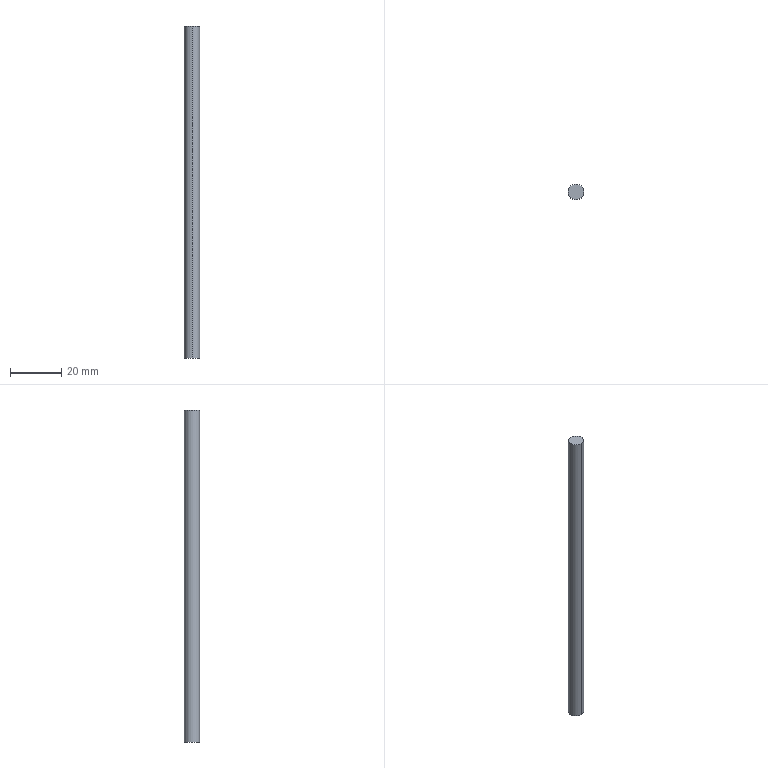Component | SolidWorks | DriveStripAxis-2 | 1 solid | 4 faces | box 6 x 6 x 130 mm | volume 3676 mm3 | cylinder 2 | plane 2 | commonest cylinder face diameters 6 x2
build123d program:
from build123d import *

# Parameters (mm, degrees)
SKETCH1_R           = 3
BOSS_EXTRUDE1_DEPTH = 130


with BuildPart() as part:
    # Sketch1 → Boss-Extrude1 (new body)
    with BuildSketch(Plane.XY):
        with Locations((71.434, 305)):
            Circle(SKETCH1_R)
    extrude(amount=-BOSS_EXTRUDE1_DEPTH)


solid = part.part

# Placed as in the assembly
solid = solid.moved(Location((-511.434, -213, 65), (0, 0, 0)))
STEP:
#1=COLOUR_RGB('',0.7922,0.8196,0.9333);
#2=FILL_AREA_STYLE_COLOUR('',#1);
#3=FILL_AREA_STYLE('',(#2));
#4=SURFACE_STYLE_FILL_AREA(#3);
#5=SURFACE_SIDE_STYLE('',(#4));
#6=SURFACE_STYLE_USAGE(.BOTH.,#5);
#7=PRESENTATION_STYLE_ASSIGNMENT((#6));
#8=CARTESIAN_POINT('',(-17.323,3.74,-2.559));
#9=VERTEX_POINT('',#8);
#10=CARTESIAN_POINT('',(-17.323,3.504,-2.559));
#11=VERTEX_POINT('',#10);
#12=CARTESIAN_POINT('',(-17.323,3.622,-2.559));
#13=DIRECTION('',(0.,0.,1.));
#14=DIRECTION('',(0.,1.,0.));
#15=AXIS2_PLACEMENT_3D('',#12,#13,#14);
#16=CIRCLE('',#15,0.1181);
#17=EDGE_CURVE('',#9,#11,#16,.T.);
#18=ORIENTED_EDGE('',*,*,#17,.T.);
#19=CARTESIAN_POINT('',(-17.323,3.504,2.559));
#20=VERTEX_POINT('',#19);
#21=CARTESIAN_POINT('',(-17.323,3.504,-2.559));
#22=DIRECTION('',(0.,0.,1.));
#23=VECTOR('',#22,39.37);
#24=LINE('',#21,#23);
#25=EDGE_CURVE('',#11,#20,#24,.T.);
#26=ORIENTED_EDGE('',*,*,#25,.T.);
#27=CARTESIAN_POINT('',(-17.323,3.74,2.559));
#28=VERTEX_POINT('',#27);
#29=CARTESIAN_POINT('',(-17.323,3.622,2.559));
#30=DIRECTION('',(0.,0.,1.));
#31=DIRECTION('',(0.,1.,0.));
#32=AXIS2_PLACEMENT_3D('',#29,#30,#31);
#33=CIRCLE('',#32,0.1181);
#34=EDGE_CURVE('',#28,#20,#33,.T.);
#35=ORIENTED_EDGE('',*,*,#34,.F.);
#36=CARTESIAN_POINT('',(-17.323,3.74,-2.559));
#37=DIRECTION('',(0.,0.,1.));
#38=VECTOR('',#37,39.37);
#39=LINE('',#36,#38);
#40=EDGE_CURVE('',#9,#28,#39,.T.);
#41=ORIENTED_EDGE('',*,*,#40,.F.);
#42=EDGE_LOOP('',(#18,#26,#35,#41));
#43=FACE_OUTER_BOUND('',#42,.T.);
#44=CARTESIAN_POINT('',(-17.323,3.622,-2.559));
#45=DIRECTION('',(0.,0.,1.));
#46=DIRECTION('',(0.,1.,0.));
#47=AXIS2_PLACEMENT_3D('',#44,#45,#46);
#48=CYLINDRICAL_SURFACE('',#47,0.1181);
#49=ADVANCED_FACE('',(#43),#48,.T.);
#50=ORIENTED_EDGE('',*,*,#25,.F.);
#51=CARTESIAN_POINT('',(-17.323,3.622,-2.559));
#52=DIRECTION('',(0.,0.,1.));
#53=DIRECTION('',(0.,1.,0.));
#54=AXIS2_PLACEMENT_3D('',#51,#52,#53);
#55=CIRCLE('',#54,0.1181);
#56=EDGE_CURVE('',#11,#9,#55,.T.);
#57=ORIENTED_EDGE('',*,*,#56,.T.);
#58=ORIENTED_EDGE('',*,*,#40,.T.);
#59=CARTESIAN_POINT('',(-17.323,3.622,2.559));
#60=DIRECTION('',(0.,0.,1.));
#61=DIRECTION('',(0.,1.,0.));
#62=AXIS2_PLACEMENT_3D('',#59,#60,#61);
#63=CIRCLE('',#62,0.1181);
#64=EDGE_CURVE('',#20,#28,#63,.T.);
#65=ORIENTED_EDGE('',*,*,#64,.F.);
#66=EDGE_LOOP('',(#50,#57,#58,#65));
#67=FACE_OUTER_BOUND('',#66,.T.);
#68=CARTESIAN_POINT('',(-17.323,3.622,-2.559));
#69=DIRECTION('',(0.,0.,1.));
#70=DIRECTION('',(0.,1.,0.));
#71=AXIS2_PLACEMENT_3D('',#68,#69,#70);
#72=CYLINDRICAL_SURFACE('',#71,0.1181);
#73=ADVANCED_FACE('',(#67),#72,.T.);
#74=ORIENTED_EDGE('',*,*,#17,.F.);
#75=ORIENTED_EDGE('',*,*,#56,.F.);
#76=EDGE_LOOP('',(#74,#75));
#77=FACE_OUTER_BOUND('',#76,.T.);
#78=CARTESIAN_POINT('',(-17.323,3.622,-2.559));
#79=DIRECTION('',(0.,0.,1.));
#80=DIRECTION('',(0.,1.,0.));
#81=AXIS2_PLACEMENT_3D('',#78,#79,#80);
#82=PLANE('',#81);
#83=ADVANCED_FACE('',(#77),#82,.F.);
#84=ORIENTED_EDGE('',*,*,#34,.T.);
#85=ORIENTED_EDGE('',*,*,#64,.T.);
#86=EDGE_LOOP('',(#84,#85));
#87=FACE_OUTER_BOUND('',#86,.T.);
#88=CARTESIAN_POINT('',(-17.323,3.622,2.559));
#89=DIRECTION('',(0.,0.,1.));
#90=DIRECTION('',(0.,1.,0.));
#91=AXIS2_PLACEMENT_3D('',#88,#89,#90);
#92=PLANE('',#91);
#93=ADVANCED_FACE('',(#87),#92,.T.);
#94=CLOSED_SHELL('',(#49,#73,#83,#93));
#95=MANIFOLD_SOLID_BREP('',#94);
#96=STYLED_ITEM('',(#7),#95);
#97=(LENGTH_UNIT()NAMED_UNIT(*)SI_UNIT($,.METRE.));
#98=LENGTH_MEASURE_WITH_UNIT(LENGTH_MEASURE(0.0254),#97);
#99=DIMENSIONAL_EXPONENTS(1.,0.,0.,0.,0.,0.,0.);
#100=(CONVERSION_BASED_UNIT('',#98)LENGTH_UNIT()NAMED_UNIT(#99));
#101=UNCERTAINTY_MEASURE_WITH_UNIT(LENGTH_MEASURE(0.00001),#100,'','');
#102=(NAMED_UNIT(*)PLANE_ANGLE_UNIT()SI_UNIT($,.RADIAN.));
#103=(NAMED_UNIT(*)SI_UNIT($,.STERADIAN.)SOLID_ANGLE_UNIT());
#104=(GEOMETRIC_REPRESENTATION_CONTEXT(3)GLOBAL_UNCERTAINTY_ASSIGNED_CONTEXT((#101))GLOBAL_UNIT_ASSIGNED_CONTEXT((#100,#102,#103))REPRESENTATION_CONTEXT('',''));
#105=MECHANICAL_DESIGN_GEOMETRIC_PRESENTATION_REPRESENTATION('',(#96),#104);
#106=PRESENTATION_LAYER_ASSIGNMENT('','',(#96));
#107=CARTESIAN_POINT('',(0.,0.,0.));
#108=DIRECTION('',(0.,0.,1.));
#109=DIRECTION('',(1.,0.,0.));
#110=AXIS2_PLACEMENT_3D('',#107,#108,#109);
#111=(LENGTH_UNIT()NAMED_UNIT(*)SI_UNIT($,.METRE.));
#112=LENGTH_MEASURE_WITH_UNIT(LENGTH_MEASURE(0.0254),#111);
#113=DIMENSIONAL_EXPONENTS(1.,0.,0.,0.,0.,0.,0.);
#114=(CONVERSION_BASED_UNIT('',#112)LENGTH_UNIT()NAMED_UNIT(#113));
#115=UNCERTAINTY_MEASURE_WITH_UNIT(LENGTH_MEASURE(0.00001),#114,'','');
#116=(NAMED_UNIT(*)PLANE_ANGLE_UNIT()SI_UNIT($,.RADIAN.));
#117=(NAMED_UNIT(*)SI_UNIT($,.STERADIAN.)SOLID_ANGLE_UNIT());
#118=(GEOMETRIC_REPRESENTATION_CONTEXT(3)GLOBAL_UNCERTAINTY_ASSIGNED_CONTEXT((#115))GLOBAL_UNIT_ASSIGNED_CONTEXT((#114,#116,#117))REPRESENTATION_CONTEXT('',''));
#119=ADVANCED_BREP_SHAPE_REPRESENTATION('',(#95,#110),#118);